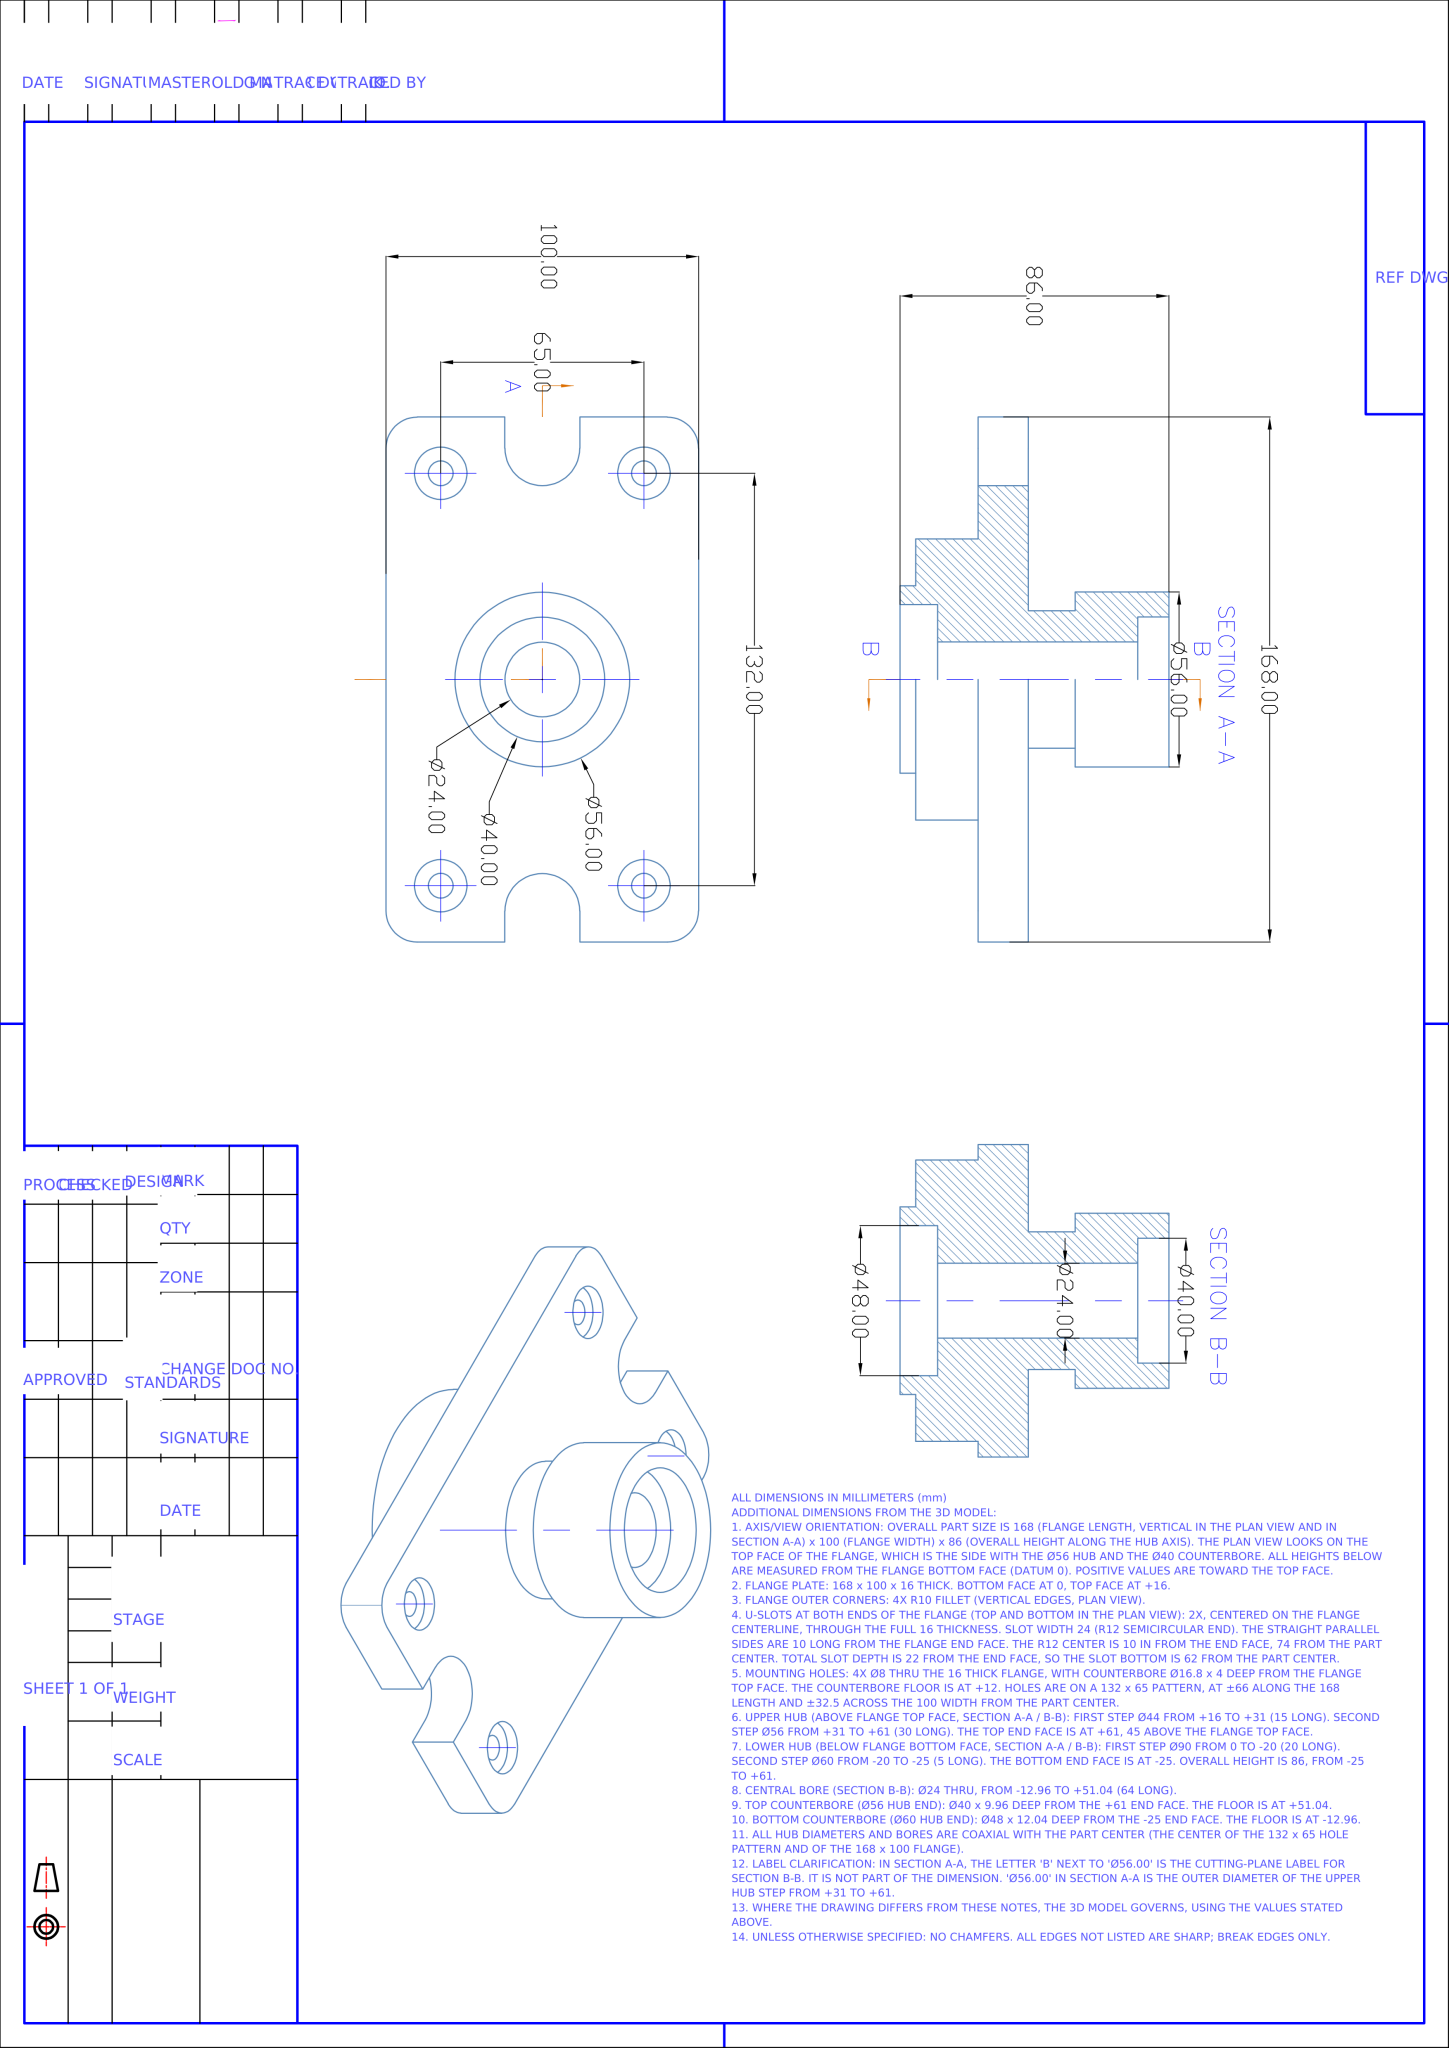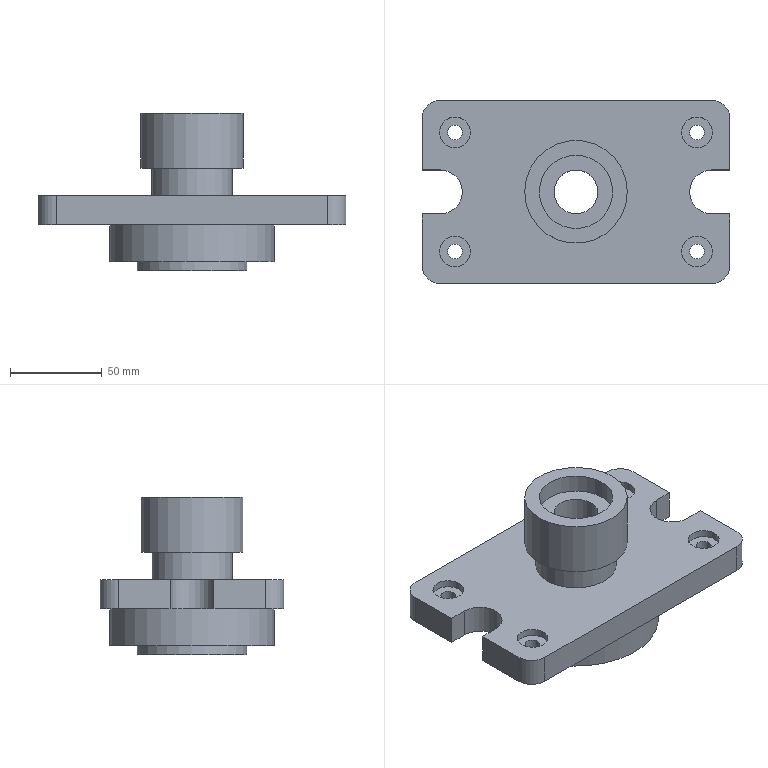Part | NX | mm | 1 solid | 43 faces | box 168 x 100 x 86 mm | volume 421364 mm3 | plane 22 | cylinder 21 | commonest cylinder face diameters 20 x4 8 x4 16.8 x4 24 x3 60 x1 90 x1 56 x1 44 x1